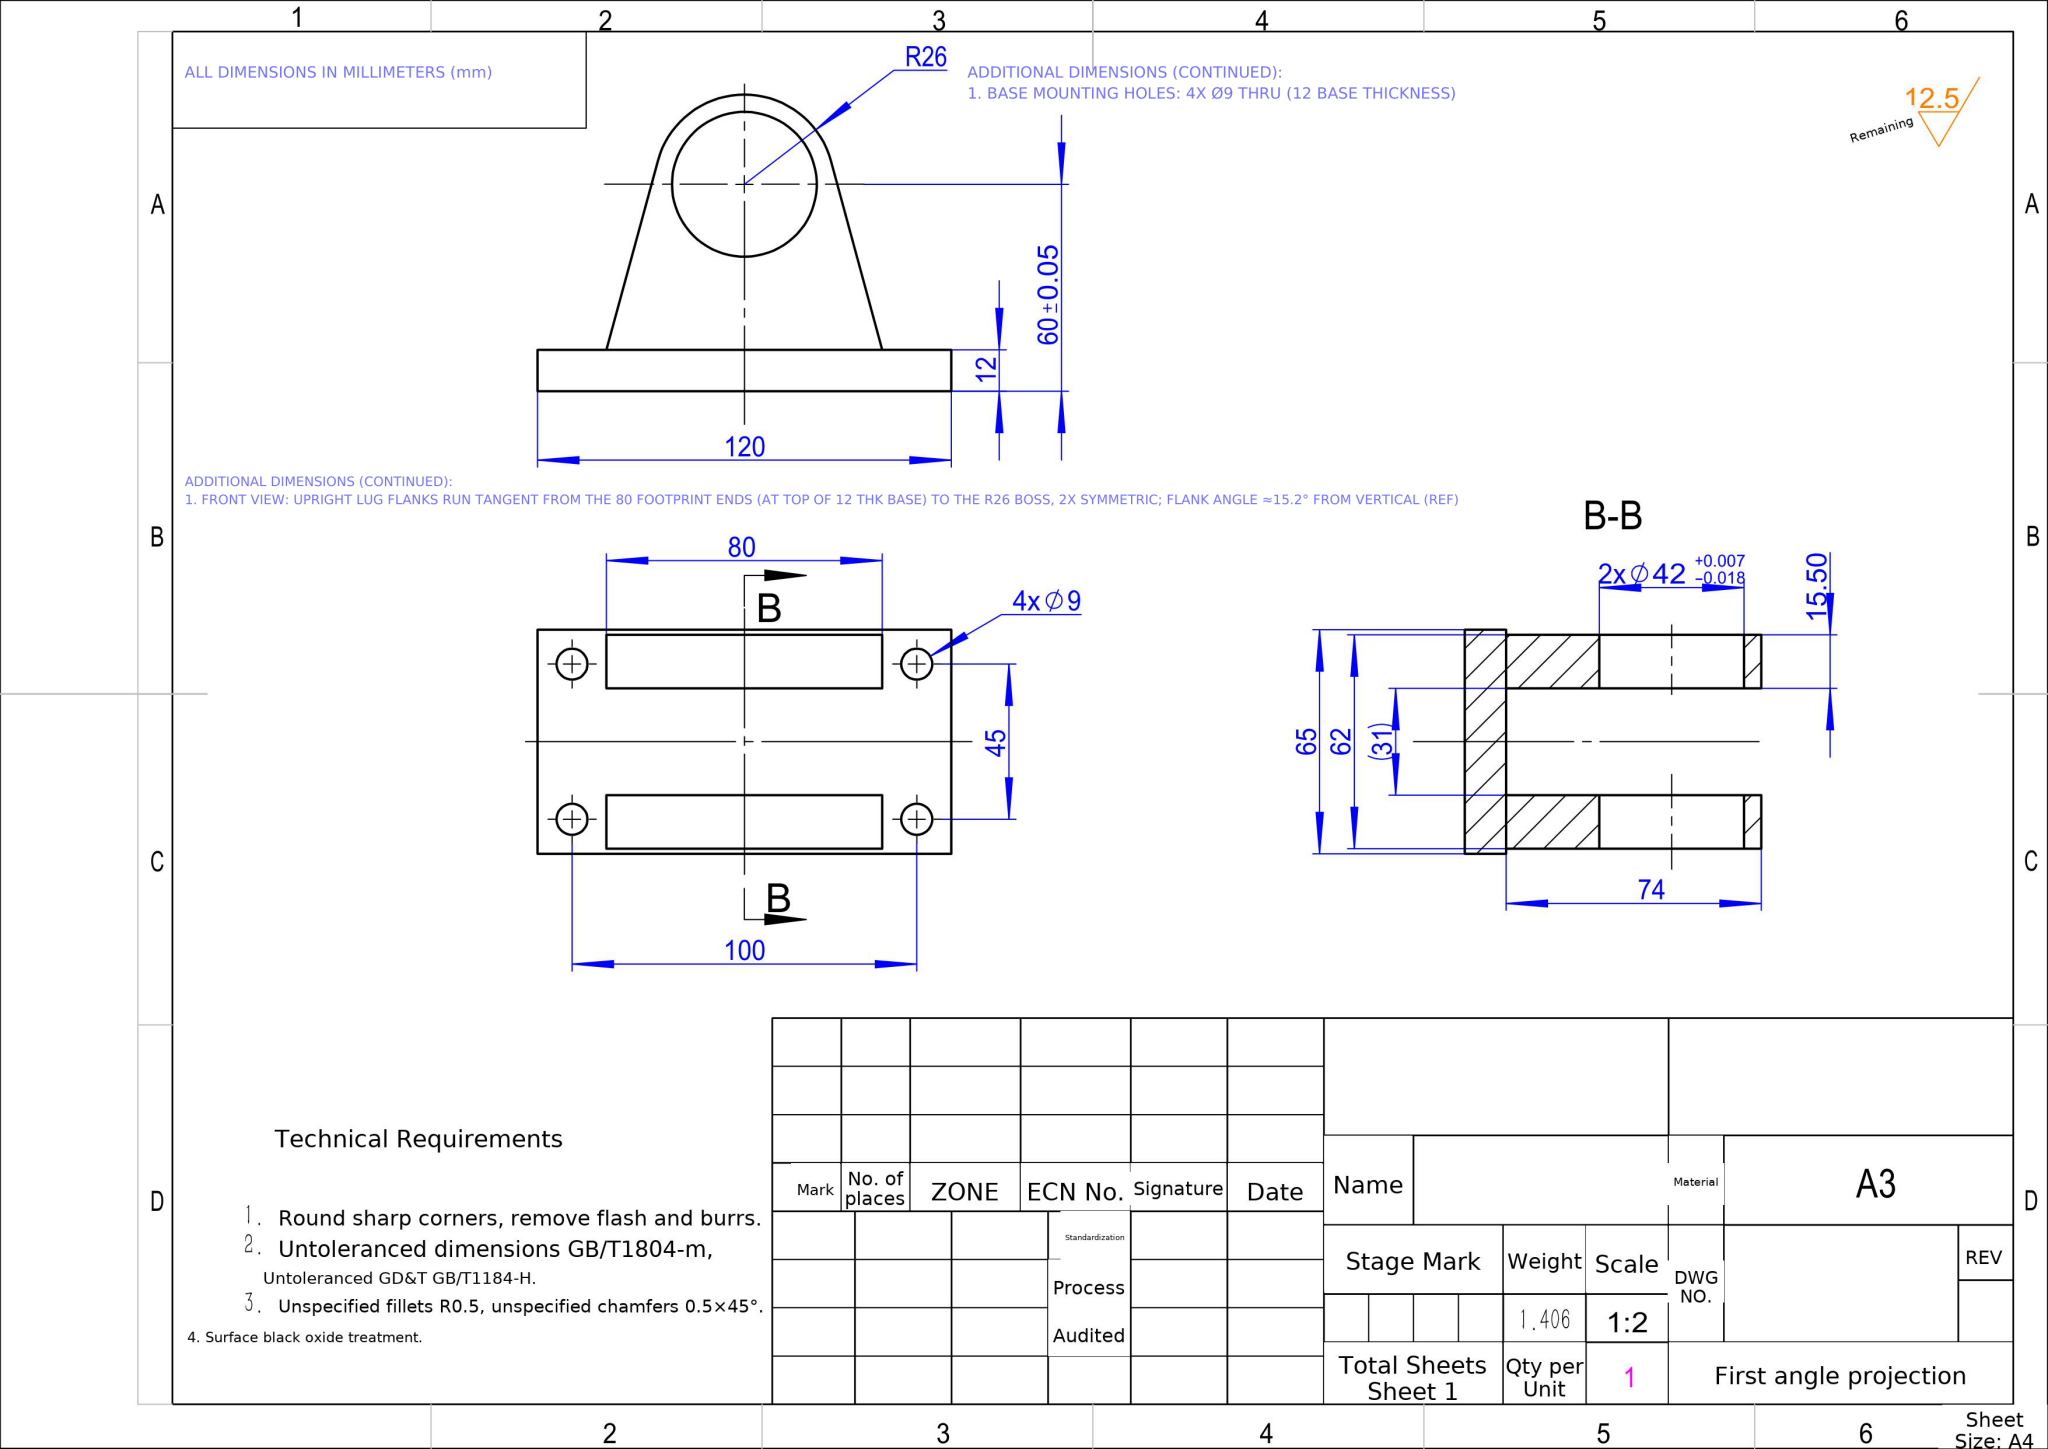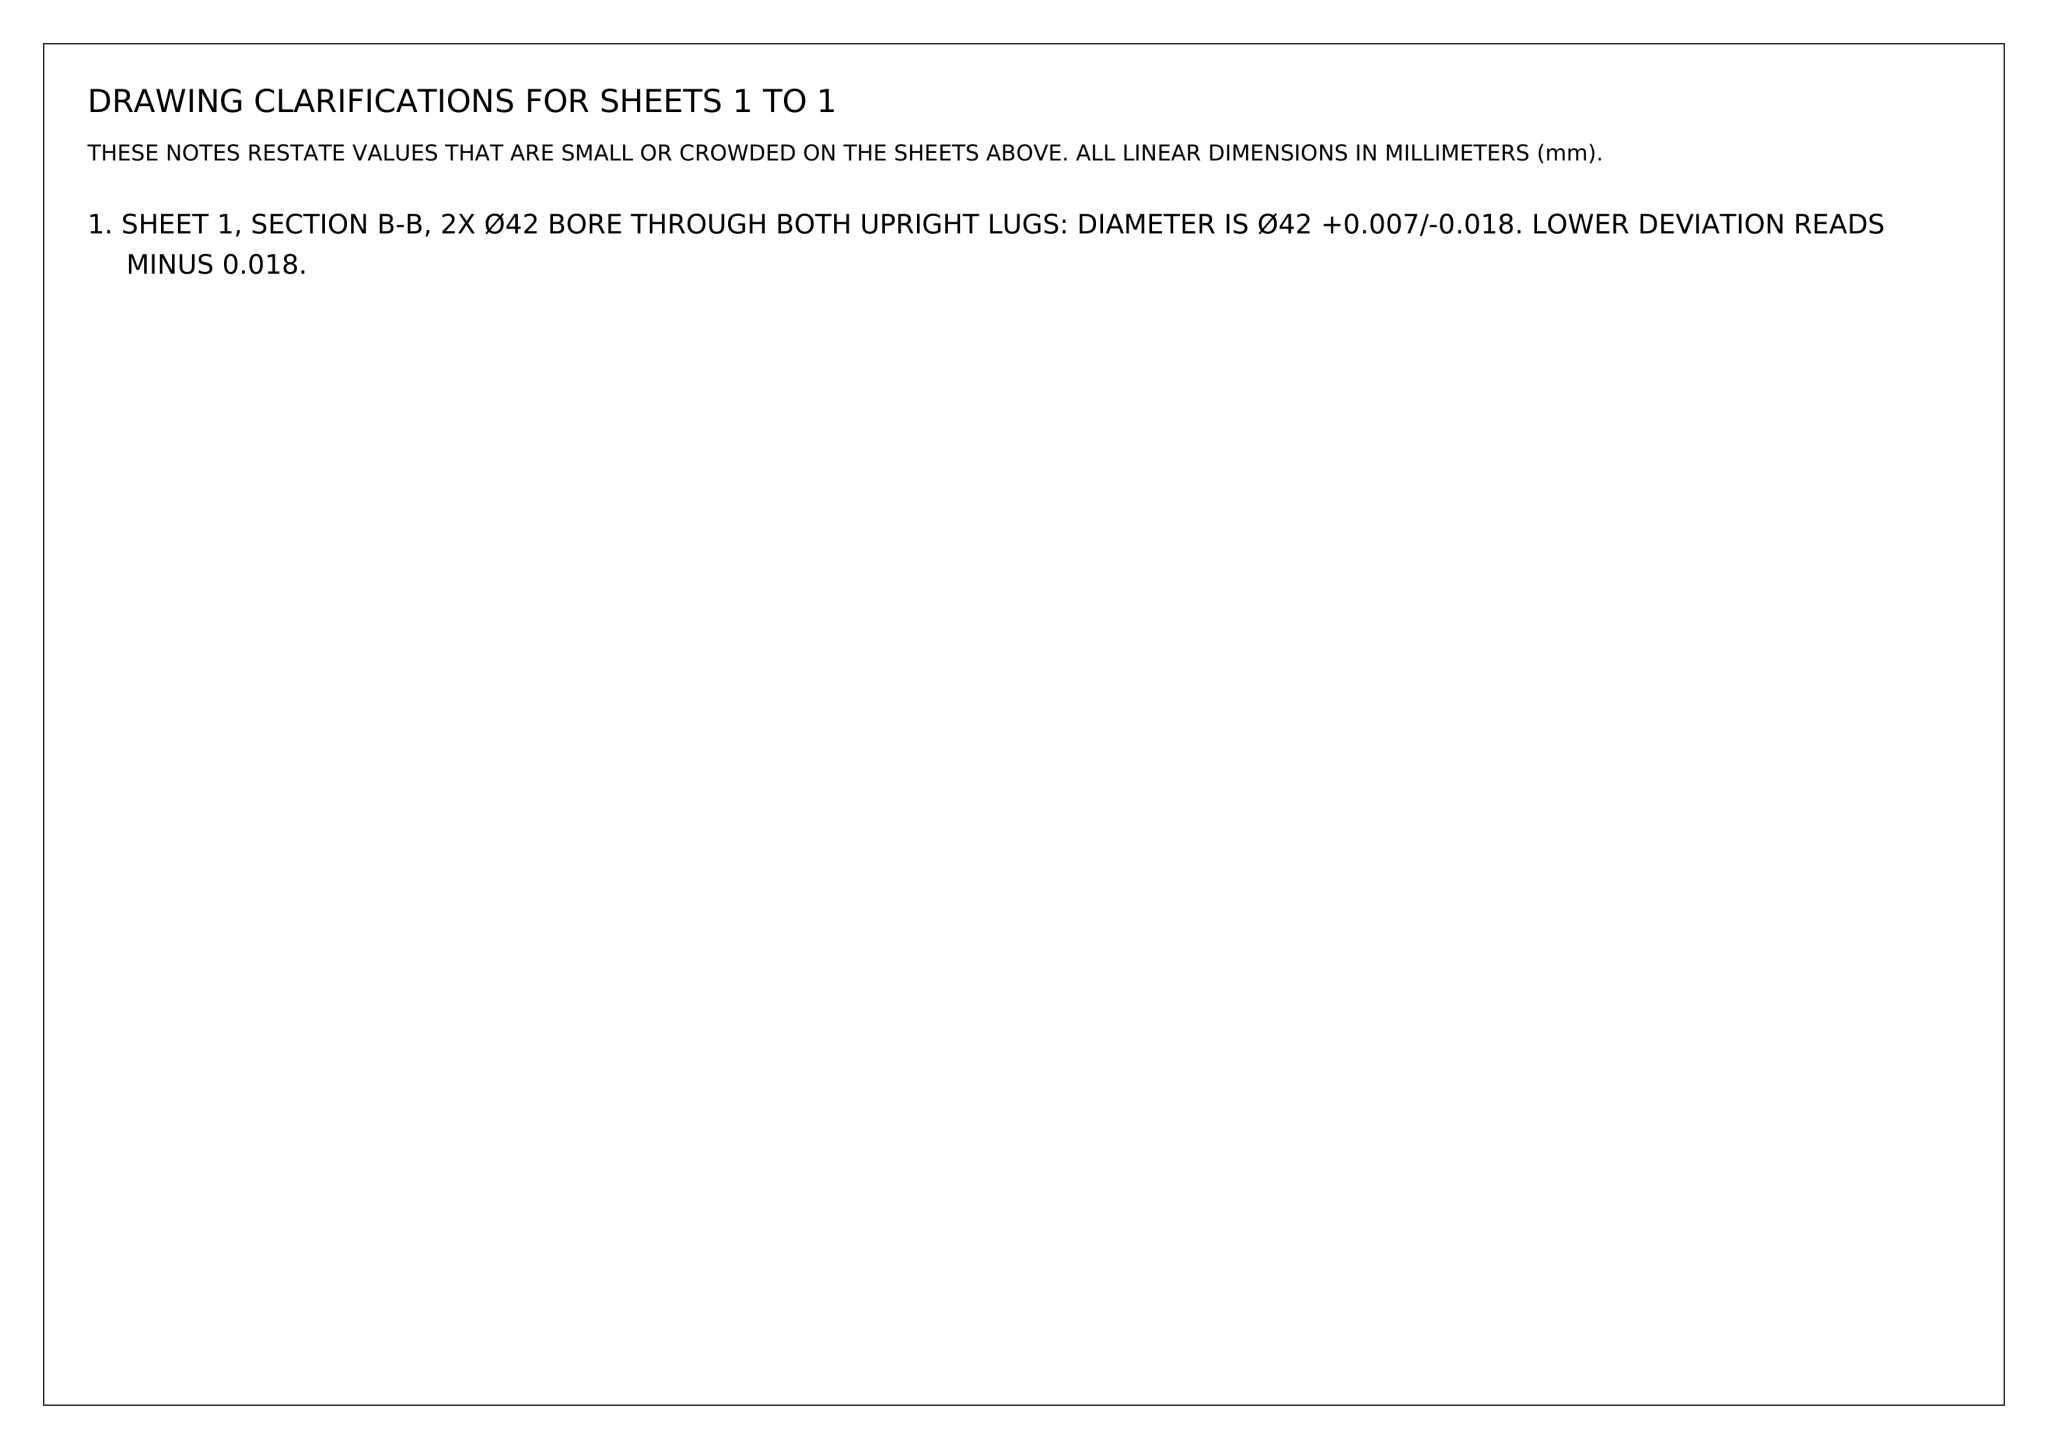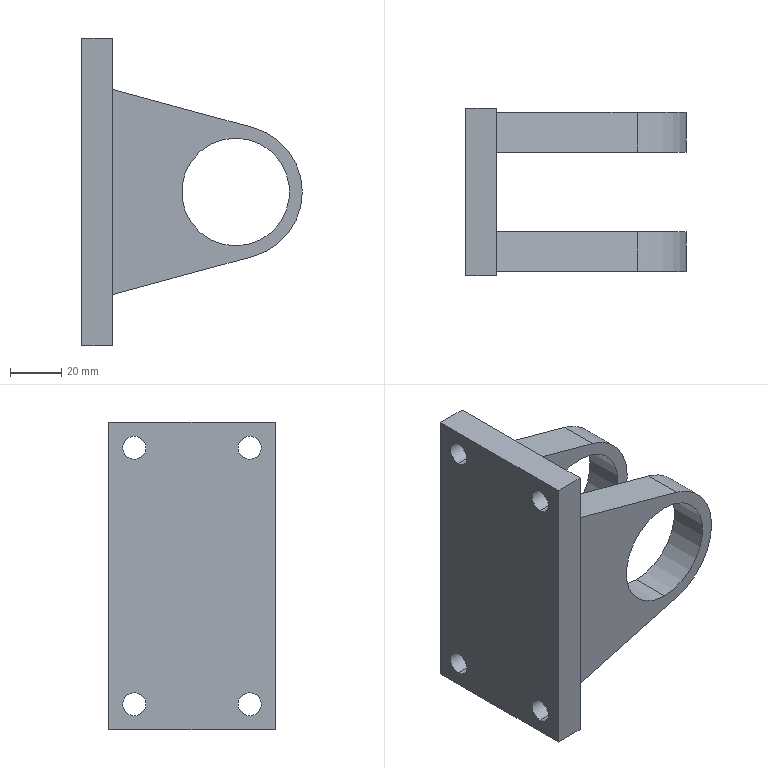Part | NX | mm | 1 solid | 28 faces | box 86 x 65 x 120 mm | volume 180263 mm3 | cylinder 14 | plane 14 | commonest cylinder face diameters 9 x8 42 x4 52 x2
STEP:
#1=COLOUR_RGB('',0.7922,0.8196,0.9333);
#2=FILL_AREA_STYLE_COLOUR('',#1);
#3=FILL_AREA_STYLE('',(#2));
#4=SURFACE_STYLE_FILL_AREA(#3);
#5=SURFACE_SIDE_STYLE('',(#4));
#6=SURFACE_STYLE_USAGE(.BOTH.,#5);
#7=PRESENTATION_STYLE_ASSIGNMENT((#6));
#8=CARTESIAN_POINT('',(60.,-15.5,-21.));
#9=VERTEX_POINT('',#8);
#10=CARTESIAN_POINT('',(60.,-31.,-21.));
#11=VERTEX_POINT('',#10);
#12=CARTESIAN_POINT('',(60.,32.5,-21.));
#13=DIRECTION('',(0.,-1.,0.));
#14=VECTOR('',#13,1000.);
#15=LINE('',#12,#14);
#16=EDGE_CURVE('',#9,#11,#15,.T.);
#17=ORIENTED_EDGE('',*,*,#16,.F.);
#18=CARTESIAN_POINT('',(60.,-15.5,21.));
#19=VERTEX_POINT('',#18);
#20=CARTESIAN_POINT('',(60.,-15.5,0.));
#21=DIRECTION('',(0.,-1.,0.));
#22=DIRECTION('',(0.,0.,-1.));
#23=AXIS2_PLACEMENT_3D('',#20,#21,#22);
#24=CIRCLE('',#23,21.);
#25=EDGE_CURVE('',#19,#9,#24,.T.);
#26=ORIENTED_EDGE('',*,*,#25,.F.);
#27=CARTESIAN_POINT('',(60.,-31.,21.));
#28=VERTEX_POINT('',#27);
#29=CARTESIAN_POINT('',(60.,32.5,21.));
#30=DIRECTION('',(0.,-1.,0.));
#31=VECTOR('',#30,1000.);
#32=LINE('',#29,#31);
#33=EDGE_CURVE('',#19,#28,#32,.T.);
#34=ORIENTED_EDGE('',*,*,#33,.T.);
#35=CARTESIAN_POINT('',(60.,-31.,0.));
#36=DIRECTION('',(0.,1.,0.));
#37=DIRECTION('',(0.,0.,1.));
#38=AXIS2_PLACEMENT_3D('',#35,#36,#37);
#39=CIRCLE('',#38,21.);
#40=EDGE_CURVE('',#11,#28,#39,.T.);
#41=ORIENTED_EDGE('',*,*,#40,.F.);
#42=EDGE_LOOP('',(#17,#26,#34,#41));
#43=FACE_OUTER_BOUND('',#42,.T.);
#44=CARTESIAN_POINT('',(60.,32.5,0.));
#45=DIRECTION('',(0.,-1.,0.));
#46=DIRECTION('',(0.,0.,1.));
#47=AXIS2_PLACEMENT_3D('',#44,#45,#46);
#48=CYLINDRICAL_SURFACE('',#47,21.);
#49=ADVANCED_FACE('',(#43),#48,.F.);
#50=CARTESIAN_POINT('',(66.824,-15.5,-25.089));
#51=VERTEX_POINT('',#50);
#52=CARTESIAN_POINT('',(12.,-15.5,-40.));
#53=VERTEX_POINT('',#52);
#54=CARTESIAN_POINT('',(12.,-15.5,-40.));
#55=DIRECTION('',(-0.9649,0.,-0.2625));
#56=VECTOR('',#55,1000.);
#57=LINE('',#54,#56);
#58=EDGE_CURVE('',#51,#53,#57,.T.);
#59=ORIENTED_EDGE('',*,*,#58,.F.);
#60=CARTESIAN_POINT('',(66.824,-31.,-25.089));
#61=VERTEX_POINT('',#60);
#62=CARTESIAN_POINT('',(66.824,-31.,-25.089));
#63=DIRECTION('',(0.,1.,0.));
#64=VECTOR('',#63,1000.);
#65=LINE('',#62,#64);
#66=EDGE_CURVE('',#61,#51,#65,.T.);
#67=ORIENTED_EDGE('',*,*,#66,.F.);
#68=CARTESIAN_POINT('',(12.,-31.,-40.));
#69=VERTEX_POINT('',#68);
#70=CARTESIAN_POINT('',(12.,-31.,-40.));
#71=DIRECTION('',(-0.9649,0.,-0.2625));
#72=VECTOR('',#71,1000.);
#73=LINE('',#70,#72);
#74=EDGE_CURVE('',#61,#69,#73,.T.);
#75=ORIENTED_EDGE('',*,*,#74,.T.);
#76=CARTESIAN_POINT('',(12.,-31.,-40.));
#77=DIRECTION('',(0.,1.,0.));
#78=VECTOR('',#77,1000.);
#79=LINE('',#76,#78);
#80=EDGE_CURVE('',#69,#53,#79,.T.);
#81=ORIENTED_EDGE('',*,*,#80,.T.);
#82=EDGE_LOOP('',(#59,#67,#75,#81));
#83=FACE_OUTER_BOUND('',#82,.T.);
#84=CARTESIAN_POINT('',(12.,-31.,-40.));
#85=DIRECTION('',(-0.2625,0.,0.9649));
#86=DIRECTION('',(0.,1.,0.));
#87=AXIS2_PLACEMENT_3D('',#84,#85,#86);
#88=PLANE('',#87);
#89=ADVANCED_FACE('',(#83),#88,.F.);
#90=CARTESIAN_POINT('',(66.824,-15.5,25.089));
#91=VERTEX_POINT('',#90);
#92=CARTESIAN_POINT('',(60.,-15.5,0.));
#93=DIRECTION('',(0.,1.,0.));
#94=DIRECTION('',(0.,0.,-1.));
#95=AXIS2_PLACEMENT_3D('',#92,#93,#94);
#96=CIRCLE('',#95,26.);
#97=EDGE_CURVE('',#91,#51,#96,.T.);
#98=ORIENTED_EDGE('',*,*,#97,.F.);
#99=CARTESIAN_POINT('',(66.824,-31.,25.089));
#100=VERTEX_POINT('',#99);
#101=CARTESIAN_POINT('',(66.824,-31.,25.089));
#102=DIRECTION('',(0.,1.,0.));
#103=VECTOR('',#102,1000.);
#104=LINE('',#101,#103);
#105=EDGE_CURVE('',#100,#91,#104,.T.);
#106=ORIENTED_EDGE('',*,*,#105,.F.);
#107=CARTESIAN_POINT('',(60.,-31.,0.));
#108=DIRECTION('',(0.,1.,0.));
#109=DIRECTION('',(0.,0.,-1.));
#110=AXIS2_PLACEMENT_3D('',#107,#108,#109);
#111=CIRCLE('',#110,26.);
#112=EDGE_CURVE('',#100,#61,#111,.T.);
#113=ORIENTED_EDGE('',*,*,#112,.T.);
#114=ORIENTED_EDGE('',*,*,#66,.T.);
#115=EDGE_LOOP('',(#98,#106,#113,#114));
#116=FACE_OUTER_BOUND('',#115,.T.);
#117=CARTESIAN_POINT('',(60.,-31.,0.));
#118=DIRECTION('',(0.,1.,0.));
#119=DIRECTION('',(0.,0.,-1.));
#120=AXIS2_PLACEMENT_3D('',#117,#118,#119);
#121=CYLINDRICAL_SURFACE('',#120,26.);
#122=ADVANCED_FACE('',(#116),#121,.T.);
#123=CARTESIAN_POINT('',(12.,-15.5,40.));
#124=VERTEX_POINT('',#123);
#125=CARTESIAN_POINT('',(66.824,-15.5,25.089));
#126=DIRECTION('',(0.9649,0.,-0.2625));
#127=VECTOR('',#126,1000.);
#128=LINE('',#125,#127);
#129=EDGE_CURVE('',#124,#91,#128,.T.);
#130=ORIENTED_EDGE('',*,*,#129,.F.);
#131=CARTESIAN_POINT('',(12.,-31.,40.));
#132=VERTEX_POINT('',#131);
#133=CARTESIAN_POINT('',(12.,-31.,40.));
#134=DIRECTION('',(0.,1.,0.));
#135=VECTOR('',#134,1000.);
#136=LINE('',#133,#135);
#137=EDGE_CURVE('',#132,#124,#136,.T.);
#138=ORIENTED_EDGE('',*,*,#137,.F.);
#139=CARTESIAN_POINT('',(66.824,-31.,25.089));
#140=DIRECTION('',(0.9649,0.,-0.2625));
#141=VECTOR('',#140,1000.);
#142=LINE('',#139,#141);
#143=EDGE_CURVE('',#132,#100,#142,.T.);
#144=ORIENTED_EDGE('',*,*,#143,.T.);
#145=ORIENTED_EDGE('',*,*,#105,.T.);
#146=EDGE_LOOP('',(#130,#138,#144,#145));
#147=FACE_OUTER_BOUND('',#146,.T.);
#148=CARTESIAN_POINT('',(66.824,-31.,25.089));
#149=DIRECTION('',(-0.2625,0.,-0.9649));
#150=DIRECTION('',(-0.9649,0.,0.2625));
#151=AXIS2_PLACEMENT_3D('',#148,#149,#150);
#152=PLANE('',#151);
#153=ADVANCED_FACE('',(#147),#152,.F.);
#154=ORIENTED_EDGE('',*,*,#25,.T.);
#155=CARTESIAN_POINT('',(60.,-15.5,0.));
#156=DIRECTION('',(0.,-1.,0.));
#157=DIRECTION('',(0.,0.,-1.));
#158=AXIS2_PLACEMENT_3D('',#155,#156,#157);
#159=CIRCLE('',#158,21.);
#160=EDGE_CURVE('',#9,#19,#159,.T.);
#161=ORIENTED_EDGE('',*,*,#160,.T.);
#162=EDGE_LOOP('',(#154,#161));
#163=FACE_BOUND('',#162,.T.);
#164=CARTESIAN_POINT('',(12.,-15.5,40.));
#165=DIRECTION('',(0.,0.,1.));
#166=VECTOR('',#165,1000.);
#167=LINE('',#164,#166);
#168=EDGE_CURVE('',#53,#124,#167,.T.);
#169=ORIENTED_EDGE('',*,*,#168,.T.);
#170=ORIENTED_EDGE('',*,*,#129,.T.);
#171=ORIENTED_EDGE('',*,*,#97,.T.);
#172=ORIENTED_EDGE('',*,*,#58,.T.);
#173=EDGE_LOOP('',(#169,#170,#171,#172));
#174=FACE_OUTER_BOUND('',#173,.T.);
#175=CARTESIAN_POINT('',(60.,-15.5,0.));
#176=DIRECTION('',(0.,1.,0.));
#177=DIRECTION('',(1.,0.,0.));
#178=AXIS2_PLACEMENT_3D('',#175,#176,#177);
#179=PLANE('',#178);
#180=ADVANCED_FACE('',(#163,#174),#179,.T.);
#181=CARTESIAN_POINT('',(60.,-31.,0.));
#182=DIRECTION('',(0.,1.,0.));
#183=DIRECTION('',(0.,0.,1.));
#184=AXIS2_PLACEMENT_3D('',#181,#182,#183);
#185=CIRCLE('',#184,21.);
#186=EDGE_CURVE('',#28,#11,#185,.T.);
#187=ORIENTED_EDGE('',*,*,#186,.T.);
#188=ORIENTED_EDGE('',*,*,#40,.T.);
#189=EDGE_LOOP('',(#187,#188));
#190=FACE_BOUND('',#189,.T.);
#191=CARTESIAN_POINT('',(12.,-31.,40.));
#192=DIRECTION('',(0.,0.,1.));
#193=VECTOR('',#192,1000.);
#194=LINE('',#191,#193);
#195=EDGE_CURVE('',#69,#132,#194,.T.);
#196=ORIENTED_EDGE('',*,*,#195,.F.);
#197=ORIENTED_EDGE('',*,*,#74,.F.);
#198=ORIENTED_EDGE('',*,*,#112,.F.);
#199=ORIENTED_EDGE('',*,*,#143,.F.);
#200=EDGE_LOOP('',(#196,#197,#198,#199));
#201=FACE_OUTER_BOUND('',#200,.T.);
#202=CARTESIAN_POINT('',(60.,-31.,0.));
#203=DIRECTION('',(0.,1.,0.));
#204=DIRECTION('',(1.,0.,0.));
#205=AXIS2_PLACEMENT_3D('',#202,#203,#204);
#206=PLANE('',#205);
#207=ADVANCED_FACE('',(#190,#201),#206,.F.);
#208=ORIENTED_EDGE('',*,*,#160,.F.);
#209=ORIENTED_EDGE('',*,*,#16,.T.);
#210=ORIENTED_EDGE('',*,*,#186,.F.);
#211=ORIENTED_EDGE('',*,*,#33,.F.);
#212=EDGE_LOOP('',(#208,#209,#210,#211));
#213=FACE_OUTER_BOUND('',#212,.T.);
#214=CARTESIAN_POINT('',(60.,32.5,0.));
#215=DIRECTION('',(0.,-1.,0.));
#216=DIRECTION('',(0.,0.,1.));
#217=AXIS2_PLACEMENT_3D('',#214,#215,#216);
#218=CYLINDRICAL_SURFACE('',#217,21.);
#219=ADVANCED_FACE('',(#213),#218,.F.);
#220=CARTESIAN_POINT('',(12.,31.,-40.));
#221=VERTEX_POINT('',#220);
#222=CARTESIAN_POINT('',(12.,15.5,-40.));
#223=VERTEX_POINT('',#222);
#224=CARTESIAN_POINT('',(12.,31.,-40.));
#225=DIRECTION('',(0.,-1.,0.));
#226=VECTOR('',#225,1000.);
#227=LINE('',#224,#226);
#228=EDGE_CURVE('',#221,#223,#227,.T.);
#229=ORIENTED_EDGE('',*,*,#228,.T.);
#230=CARTESIAN_POINT('',(12.,15.5,40.));
#231=VERTEX_POINT('',#230);
#232=CARTESIAN_POINT('',(12.,15.5,40.));
#233=DIRECTION('',(0.,0.,1.));
#234=VECTOR('',#233,1000.);
#235=LINE('',#232,#234);
#236=EDGE_CURVE('',#223,#231,#235,.T.);
#237=ORIENTED_EDGE('',*,*,#236,.T.);
#238=CARTESIAN_POINT('',(12.,31.,40.));
#239=VERTEX_POINT('',#238);
#240=CARTESIAN_POINT('',(12.,31.,40.));
#241=DIRECTION('',(0.,-1.,0.));
#242=VECTOR('',#241,1000.);
#243=LINE('',#240,#242);
#244=EDGE_CURVE('',#239,#231,#243,.T.);
#245=ORIENTED_EDGE('',*,*,#244,.F.);
#246=CARTESIAN_POINT('',(12.,31.,40.));
#247=DIRECTION('',(0.,0.,1.));
#248=VECTOR('',#247,1000.);
#249=LINE('',#246,#248);
#250=EDGE_CURVE('',#221,#239,#249,.T.);
#251=ORIENTED_EDGE('',*,*,#250,.F.);
#252=EDGE_LOOP('',(#229,#237,#245,#251));
#253=FACE_BOUND('',#252,.T.);
#254=CARTESIAN_POINT('',(12.,-32.5,-60.));
#255=VERTEX_POINT('',#254);
#256=CARTESIAN_POINT('',(12.,32.5,-60.));
#257=VERTEX_POINT('',#256);
#258=CARTESIAN_POINT('',(12.,32.5,-60.));
#259=DIRECTION('',(0.,1.,0.));
#260=VECTOR('',#259,1000.);
#261=LINE('',#258,#260);
#262=EDGE_CURVE('',#255,#257,#261,.T.);
#263=ORIENTED_EDGE('',*,*,#262,.T.);
#264=CARTESIAN_POINT('',(12.,32.5,60.));
#265=VERTEX_POINT('',#264);
#266=CARTESIAN_POINT('',(12.,32.5,60.));
#267=DIRECTION('',(0.,0.,1.));
#268=VECTOR('',#267,1000.);
#269=LINE('',#266,#268);
#270=EDGE_CURVE('',#257,#265,#269,.T.);
#271=ORIENTED_EDGE('',*,*,#270,.T.);
#272=CARTESIAN_POINT('',(12.,-32.5,60.));
#273=VERTEX_POINT('',#272);
#274=CARTESIAN_POINT('',(12.,32.5,60.));
#275=DIRECTION('',(0.,-1.,0.));
#276=VECTOR('',#275,1000.);
#277=LINE('',#274,#276);
#278=EDGE_CURVE('',#265,#273,#277,.T.);
#279=ORIENTED_EDGE('',*,*,#278,.T.);
#280=CARTESIAN_POINT('',(12.,-32.5,60.));
#281=DIRECTION('',(0.,0.,-1.));
#282=VECTOR('',#281,1000.);
#283=LINE('',#280,#282);
#284=EDGE_CURVE('',#273,#255,#283,.T.);
#285=ORIENTED_EDGE('',*,*,#284,.T.);
#286=EDGE_LOOP('',(#263,#271,#279,#285));
#287=FACE_OUTER_BOUND('',#286,.T.);
#288=CARTESIAN_POINT('',(12.,22.5,45.5));
#289=VERTEX_POINT('',#288);
#290=CARTESIAN_POINT('',(12.,22.5,54.5));
#291=VERTEX_POINT('',#290);
#292=CARTESIAN_POINT('',(12.,22.5,50.));
#293=DIRECTION('',(1.,0.,0.));
#294=DIRECTION('',(0.,0.,-1.));
#295=AXIS2_PLACEMENT_3D('',#292,#293,#294);
#296=CIRCLE('',#295,4.5);
#297=EDGE_CURVE('',#289,#291,#296,.T.);
#298=ORIENTED_EDGE('',*,*,#297,.F.);
#299=CARTESIAN_POINT('',(12.,22.5,50.));
#300=DIRECTION('',(1.,0.,0.));
#301=DIRECTION('',(0.,0.,-1.));
#302=AXIS2_PLACEMENT_3D('',#299,#300,#301);
#303=CIRCLE('',#302,4.5);
#304=EDGE_CURVE('',#291,#289,#303,.T.);
#305=ORIENTED_EDGE('',*,*,#304,.F.);
#306=EDGE_LOOP('',(#298,#305));
#307=FACE_BOUND('',#306,.T.);
#308=CARTESIAN_POINT('',(12.,-22.5,45.5));
#309=VERTEX_POINT('',#308);
#310=CARTESIAN_POINT('',(12.,-22.5,54.5));
#311=VERTEX_POINT('',#310);
#312=CARTESIAN_POINT('',(12.,-22.5,50.));
#313=DIRECTION('',(1.,0.,0.));
#314=DIRECTION('',(0.,0.,-1.));
#315=AXIS2_PLACEMENT_3D('',#312,#313,#314);
#316=CIRCLE('',#315,4.5);
#317=EDGE_CURVE('',#309,#311,#316,.T.);
#318=ORIENTED_EDGE('',*,*,#317,.F.);
#319=CARTESIAN_POINT('',(12.,-22.5,50.));
#320=DIRECTION('',(1.,0.,0.));
#321=DIRECTION('',(0.,0.,-1.));
#322=AXIS2_PLACEMENT_3D('',#319,#320,#321);
#323=CIRCLE('',#322,4.5);
#324=EDGE_CURVE('',#311,#309,#323,.T.);
#325=ORIENTED_EDGE('',*,*,#324,.F.);
#326=EDGE_LOOP('',(#318,#325));
#327=FACE_BOUND('',#326,.T.);
#328=CARTESIAN_POINT('',(12.,-22.5,-54.5));
#329=VERTEX_POINT('',#328);
#330=CARTESIAN_POINT('',(12.,-22.5,-45.5));
#331=VERTEX_POINT('',#330);
#332=CARTESIAN_POINT('',(12.,-22.5,-50.));
#333=DIRECTION('',(1.,0.,0.));
#334=DIRECTION('',(0.,0.,-1.));
#335=AXIS2_PLACEMENT_3D('',#332,#333,#334);
#336=CIRCLE('',#335,4.5);
#337=EDGE_CURVE('',#329,#331,#336,.T.);
#338=ORIENTED_EDGE('',*,*,#337,.F.);
#339=CARTESIAN_POINT('',(12.,-22.5,-50.));
#340=DIRECTION('',(1.,0.,0.));
#341=DIRECTION('',(0.,0.,-1.));
#342=AXIS2_PLACEMENT_3D('',#339,#340,#341);
#343=CIRCLE('',#342,4.5);
#344=EDGE_CURVE('',#331,#329,#343,.T.);
#345=ORIENTED_EDGE('',*,*,#344,.F.);
#346=EDGE_LOOP('',(#338,#345));
#347=FACE_BOUND('',#346,.T.);
#348=CARTESIAN_POINT('',(12.,22.5,-54.5));
#349=VERTEX_POINT('',#348);
#350=CARTESIAN_POINT('',(12.,22.5,-45.5));
#351=VERTEX_POINT('',#350);
#352=CARTESIAN_POINT('',(12.,22.5,-50.));
#353=DIRECTION('',(1.,0.,0.));
#354=DIRECTION('',(0.,0.,-1.));
#355=AXIS2_PLACEMENT_3D('',#352,#353,#354);
#356=CIRCLE('',#355,4.5);
#357=EDGE_CURVE('',#349,#351,#356,.T.);
#358=ORIENTED_EDGE('',*,*,#357,.F.);
#359=CARTESIAN_POINT('',(12.,22.5,-50.));
#360=DIRECTION('',(1.,0.,0.));
#361=DIRECTION('',(0.,0.,-1.));
#362=AXIS2_PLACEMENT_3D('',#359,#360,#361);
#363=CIRCLE('',#362,4.5);
#364=EDGE_CURVE('',#351,#349,#363,.T.);
#365=ORIENTED_EDGE('',*,*,#364,.F.);
#366=EDGE_LOOP('',(#358,#365));
#367=FACE_BOUND('',#366,.T.);
#368=ORIENTED_EDGE('',*,*,#168,.F.);
#369=ORIENTED_EDGE('',*,*,#80,.F.);
#370=ORIENTED_EDGE('',*,*,#195,.T.);
#371=ORIENTED_EDGE('',*,*,#137,.T.);
#372=EDGE_LOOP('',(#368,#369,#370,#371));
#373=FACE_BOUND('',#372,.T.);
#374=CARTESIAN_POINT('',(12.,0.,0.));
#375=DIRECTION('',(1.,0.,0.));
#376=DIRECTION('',(0.,1.,0.));
#377=AXIS2_PLACEMENT_3D('',#374,#375,#376);
#378=PLANE('',#377);
#379=ADVANCED_FACE('',(#253,#287,#307,#327,#347,#367,#373),#378,.T.);
#380=CARTESIAN_POINT('',(0.,22.5,54.5));
#381=VERTEX_POINT('',#380);
#382=CARTESIAN_POINT('',(12.,22.5,54.5));
#383=DIRECTION('',(1.,0.,0.));
#384=VECTOR('',#383,1000.);
#385=LINE('',#382,#384);
#386=EDGE_CURVE('',#381,#291,#385,.T.);
#387=ORIENTED_EDGE('',*,*,#386,.F.);
#388=CARTESIAN_POINT('',(0.,22.5,45.5));
#389=VERTEX_POINT('',#388);
#390=CARTESIAN_POINT('',(0.,22.5,50.));
#391=DIRECTION('',(1.,0.,0.));
#392=DIRECTION('',(0.,0.,-1.));
#393=AXIS2_PLACEMENT_3D('',#390,#391,#392);
#394=CIRCLE('',#393,4.5);
#395=EDGE_CURVE('',#389,#381,#394,.T.);
#396=ORIENTED_EDGE('',*,*,#395,.F.);
#397=CARTESIAN_POINT('',(12.,22.5,45.5));
#398=DIRECTION('',(1.,0.,0.));
#399=VECTOR('',#398,1000.);
#400=LINE('',#397,#399);
#401=EDGE_CURVE('',#389,#289,#400,.T.);
#402=ORIENTED_EDGE('',*,*,#401,.T.);
#403=ORIENTED_EDGE('',*,*,#297,.T.);
#404=EDGE_LOOP('',(#387,#396,#402,#403));
#405=FACE_OUTER_BOUND('',#404,.T.);
#406=CARTESIAN_POINT('',(12.,22.5,50.));
#407=DIRECTION('',(1.,0.,0.));
#408=DIRECTION('',(0.,0.,-1.));
#409=AXIS2_PLACEMENT_3D('',#406,#407,#408);
#410=CYLINDRICAL_SURFACE('',#409,4.5);
#411=ADVANCED_FACE('',(#405),#410,.F.);
#412=CARTESIAN_POINT('',(0.,-22.5,54.5));
#413=VERTEX_POINT('',#412);
#414=CARTESIAN_POINT('',(12.,-22.5,54.5));
#415=DIRECTION('',(1.,0.,0.));
#416=VECTOR('',#415,1000.);
#417=LINE('',#414,#416);
#418=EDGE_CURVE('',#413,#311,#417,.T.);
#419=ORIENTED_EDGE('',*,*,#418,.F.);
#420=CARTESIAN_POINT('',(0.,-22.5,45.5));
#421=VERTEX_POINT('',#420);
#422=CARTESIAN_POINT('',(0.,-22.5,50.));
#423=DIRECTION('',(1.,0.,0.));
#424=DIRECTION('',(0.,0.,-1.));
#425=AXIS2_PLACEMENT_3D('',#422,#423,#424);
#426=CIRCLE('',#425,4.5);
#427=EDGE_CURVE('',#421,#413,#426,.T.);
#428=ORIENTED_EDGE('',*,*,#427,.F.);
#429=CARTESIAN_POINT('',(12.,-22.5,45.5));
#430=DIRECTION('',(1.,0.,0.));
#431=VECTOR('',#430,1000.);
#432=LINE('',#429,#431);
#433=EDGE_CURVE('',#421,#309,#432,.T.);
#434=ORIENTED_EDGE('',*,*,#433,.T.);
#435=ORIENTED_EDGE('',*,*,#317,.T.);
#436=EDGE_LOOP('',(#419,#428,#434,#435));
#437=FACE_OUTER_BOUND('',#436,.T.);
#438=CARTESIAN_POINT('',(12.,-22.5,50.));
#439=DIRECTION('',(1.,0.,0.));
#440=DIRECTION('',(0.,0.,-1.));
#441=AXIS2_PLACEMENT_3D('',#438,#439,#440);
#442=CYLINDRICAL_SURFACE('',#441,4.5);
#443=ADVANCED_FACE('',(#437),#442,.F.);
#444=CARTESIAN_POINT('',(0.,-22.5,-45.5));
#445=VERTEX_POINT('',#444);
#446=CARTESIAN_POINT('',(12.,-22.5,-45.5));
#447=DIRECTION('',(1.,0.,0.));
#448=VECTOR('',#447,1000.);
#449=LINE('',#446,#448);
#450=EDGE_CURVE('',#445,#331,#449,.T.);
#451=ORIENTED_EDGE('',*,*,#450,.F.);
#452=CARTESIAN_POINT('',(0.,-22.5,-54.5));
#453=VERTEX_POINT('',#452);
#454=CARTESIAN_POINT('',(0.,-22.5,-50.));
#455=DIRECTION('',(1.,0.,0.));
#456=DIRECTION('',(0.,0.,-1.));
#457=AXIS2_PLACEMENT_3D('',#454,#455,#456);
#458=CIRCLE('',#457,4.5);
#459=EDGE_CURVE('',#453,#445,#458,.T.);
#460=ORIENTED_EDGE('',*,*,#459,.F.);
#461=CARTESIAN_POINT('',(12.,-22.5,-54.5));
#462=DIRECTION('',(1.,0.,0.));
#463=VECTOR('',#462,1000.);
#464=LINE('',#461,#463);
#465=EDGE_CURVE('',#453,#329,#464,.T.);
#466=ORIENTED_EDGE('',*,*,#465,.T.);
#467=ORIENTED_EDGE('',*,*,#337,.T.);
#468=EDGE_LOOP('',(#451,#460,#466,#467));
#469=FACE_OUTER_BOUND('',#468,.T.);
#470=CARTESIAN_POINT('',(12.,-22.5,-50.));
#471=DIRECTION('',(1.,0.,0.));
#472=DIRECTION('',(0.,0.,-1.));
#473=AXIS2_PLACEMENT_3D('',#470,#471,#472);
#474=CYLINDRICAL_SURFACE('',#473,4.5);
#475=ADVANCED_FACE('',(#469),#474,.F.);
#476=CARTESIAN_POINT('',(0.,22.5,-45.5));
#477=VERTEX_POINT('',#476);
#478=CARTESIAN_POINT('',(12.,22.5,-45.5));
#479=DIRECTION('',(1.,0.,0.));
#480=VECTOR('',#479,1000.);
#481=LINE('',#478,#480);
#482=EDGE_CURVE('',#477,#351,#481,.T.);
#483=ORIENTED_EDGE('',*,*,#482,.F.);
#484=CARTESIAN_POINT('',(0.,22.5,-54.5));
#485=VERTEX_POINT('',#484);
#486=CARTESIAN_POINT('',(0.,22.5,-50.));
#487=DIRECTION('',(1.,0.,0.));
#488=DIRECTION('',(0.,0.,-1.));
#489=AXIS2_PLACEMENT_3D('',#486,#487,#488);
#490=CIRCLE('',#489,4.5);
#491=EDGE_CURVE('',#485,#477,#490,.T.);
#492=ORIENTED_EDGE('',*,*,#491,.F.);
#493=CARTESIAN_POINT('',(12.,22.5,-54.5));
#494=DIRECTION('',(1.,0.,0.));
#495=VECTOR('',#494,1000.);
#496=LINE('',#493,#495);
#497=EDGE_CURVE('',#485,#349,#496,.T.);
#498=ORIENTED_EDGE('',*,*,#497,.T.);
#499=ORIENTED_EDGE('',*,*,#357,.T.);
#500=EDGE_LOOP('',(#483,#492,#498,#499));
#501=FACE_OUTER_BOUND('',#500,.T.);
#502=CARTESIAN_POINT('',(12.,22.5,-50.));
#503=DIRECTION('',(1.,0.,0.));
#504=DIRECTION('',(0.,0.,-1.));
#505=AXIS2_PLACEMENT_3D('',#502,#503,#504);
#506=CYLINDRICAL_SURFACE('',#505,4.5);
#507=ADVANCED_FACE('',(#501),#506,.F.);
#508=ORIENTED_EDGE('',*,*,#491,.T.);
#509=CARTESIAN_POINT('',(0.,22.5,-50.));
#510=DIRECTION('',(1.,0.,0.));
#511=DIRECTION('',(0.,0.,-1.));
#512=AXIS2_PLACEMENT_3D('',#509,#510,#511);
#513=CIRCLE('',#512,4.5);
#514=EDGE_CURVE('',#477,#485,#513,.T.);
#515=ORIENTED_EDGE('',*,*,#514,.T.);
#516=EDGE_LOOP('',(#508,#515));
#517=FACE_BOUND('',#516,.T.);
#518=ORIENTED_EDGE('',*,*,#459,.T.);
#519=CARTESIAN_POINT('',(0.,-22.5,-50.));
#520=DIRECTION('',(1.,0.,0.));
#521=DIRECTION('',(0.,0.,-1.));
#522=AXIS2_PLACEMENT_3D('',#519,#520,#521);
#523=CIRCLE('',#522,4.5);
#524=EDGE_CURVE('',#445,#453,#523,.T.);
#525=ORIENTED_EDGE('',*,*,#524,.T.);
#526=EDGE_LOOP('',(#518,#525));
#527=FACE_BOUND('',#526,.T.);
#528=ORIENTED_EDGE('',*,*,#427,.T.);
#529=CARTESIAN_POINT('',(0.,-22.5,50.));
#530=DIRECTION('',(1.,0.,0.));
#531=DIRECTION('',(0.,0.,-1.));
#532=AXIS2_PLACEMENT_3D('',#529,#530,#531);
#533=CIRCLE('',#532,4.5);
#534=EDGE_CURVE('',#413,#421,#533,.T.);
#535=ORIENTED_EDGE('',*,*,#534,.T.);
#536=EDGE_LOOP('',(#528,#535));
#537=FACE_BOUND('',#536,.T.);
#538=ORIENTED_EDGE('',*,*,#395,.T.);
#539=CARTESIAN_POINT('',(0.,22.5,50.));
#540=DIRECTION('',(1.,0.,0.));
#541=DIRECTION('',(0.,0.,-1.));
#542=AXIS2_PLACEMENT_3D('',#539,#540,#541);
#543=CIRCLE('',#542,4.5);
#544=EDGE_CURVE('',#381,#389,#543,.T.);
#545=ORIENTED_EDGE('',*,*,#544,.T.);
#546=EDGE_LOOP('',(#538,#545));
#547=FACE_BOUND('',#546,.T.);
#548=CARTESIAN_POINT('',(0.,-32.5,-60.));
#549=VERTEX_POINT('',#548);
#550=CARTESIAN_POINT('',(0.,32.5,-60.));
#551=VERTEX_POINT('',#550);
#552=CARTESIAN_POINT('',(0.,32.5,-60.));
#553=DIRECTION('',(0.,1.,0.));
#554=VECTOR('',#553,1000.);
#555=LINE('',#552,#554);
#556=EDGE_CURVE('',#549,#551,#555,.T.);
#557=ORIENTED_EDGE('',*,*,#556,.F.);
#558=CARTESIAN_POINT('',(0.,-32.5,60.));
#559=VERTEX_POINT('',#558);
#560=CARTESIAN_POINT('',(0.,-32.5,60.));
#561=DIRECTION('',(0.,0.,-1.));
#562=VECTOR('',#561,1000.);
#563=LINE('',#560,#562);
#564=EDGE_CURVE('',#559,#549,#563,.T.);
#565=ORIENTED_EDGE('',*,*,#564,.F.);
#566=CARTESIAN_POINT('',(0.,32.5,60.));
#567=VERTEX_POINT('',#566);
#568=CARTESIAN_POINT('',(0.,32.5,60.));
#569=DIRECTION('',(0.,-1.,0.));
#570=VECTOR('',#569,1000.);
#571=LINE('',#568,#570);
#572=EDGE_CURVE('',#567,#559,#571,.T.);
#573=ORIENTED_EDGE('',*,*,#572,.F.);
#574=CARTESIAN_POINT('',(0.,32.5,60.));
#575=DIRECTION('',(0.,0.,1.));
#576=VECTOR('',#575,1000.);
#577=LINE('',#574,#576);
#578=EDGE_CURVE('',#551,#567,#577,.T.);
#579=ORIENTED_EDGE('',*,*,#578,.F.);
#580=EDGE_LOOP('',(#557,#565,#573,#579));
#581=FACE_OUTER_BOUND('',#580,.T.);
#582=CARTESIAN_POINT('',(0.,0.,0.));
#583=DIRECTION('',(1.,0.,0.));
#584=DIRECTION('',(0.,1.,0.));
#585=AXIS2_PLACEMENT_3D('',#582,#583,#584);
#586=PLANE('',#585);
#587=ADVANCED_FACE('',(#517,#527,#537,#547,#581),#586,.F.);
#588=ORIENTED_EDGE('',*,*,#564,.T.);
#589=CARTESIAN_POINT('',(12.,-32.5,-60.));
#590=DIRECTION('',(-1.,0.,0.));
#591=VECTOR('',#590,1000.);
#592=LINE('',#589,#591);
#593=EDGE_CURVE('',#255,#549,#592,.T.);
#594=ORIENTED_EDGE('',*,*,#593,.F.);
#595=ORIENTED_EDGE('',*,*,#284,.F.);
#596=CARTESIAN_POINT('',(12.,-32.5,60.));
#597=DIRECTION('',(-1.,0.,0.));
#598=VECTOR('',#597,1000.);
#599=LINE('',#596,#598);
#600=EDGE_CURVE('',#273,#559,#599,.T.);
#601=ORIENTED_EDGE('',*,*,#600,.T.);
#602=EDGE_LOOP('',(#588,#594,#595,#601));
#603=FACE_OUTER_BOUND('',#602,.T.);
#604=CARTESIAN_POINT('',(12.,-32.5,60.));
#605=DIRECTION('',(0.,1.,0.));
#606=DIRECTION('',(1.,0.,0.));
#607=AXIS2_PLACEMENT_3D('',#604,#605,#606);
#608=PLANE('',#607);
#609=ADVANCED_FACE('',(#603),#608,.F.);
#610=ORIENTED_EDGE('',*,*,#572,.T.);
#611=ORIENTED_EDGE('',*,*,#600,.F.);
#612=ORIENTED_EDGE('',*,*,#278,.F.);
#613=CARTESIAN_POINT('',(12.,32.5,60.));
#614=DIRECTION('',(-1.,0.,0.));
#615=VECTOR('',#614,1000.);
#616=LINE('',#613,#615);
#617=EDGE_CURVE('',#265,#567,#616,.T.);
#618=ORIENTED_EDGE('',*,*,#617,.T.);
#619=EDGE_LOOP('',(#610,#611,#612,#618));
#620=FACE_OUTER_BOUND('',#619,.T.);
#621=CARTESIAN_POINT('',(12.,32.5,60.));
#622=DIRECTION('',(0.,0.,-1.));
#623=DIRECTION('',(0.,-1.,0.));
#624=AXIS2_PLACEMENT_3D('',#621,#622,#623);
#625=PLANE('',#624);
#626=ADVANCED_FACE('',(#620),#625,.F.);
#627=ORIENTED_EDGE('',*,*,#578,.T.);
#628=ORIENTED_EDGE('',*,*,#617,.F.);
#629=ORIENTED_EDGE('',*,*,#270,.F.);
#630=CARTESIAN_POINT('',(12.,32.5,-60.));
#631=DIRECTION('',(-1.,0.,0.));
#632=VECTOR('',#631,1000.);
#633=LINE('',#630,#632);
#634=EDGE_CURVE('',#257,#551,#633,.T.);
#635=ORIENTED_EDGE('',*,*,#634,.T.);
#636=EDGE_LOOP('',(#627,#628,#629,#635));
#637=FACE_OUTER_BOUND('',#636,.T.);
#638=CARTESIAN_POINT('',(12.,32.5,60.));
#639=DIRECTION('',(0.,-1.,0.));
#640=DIRECTION('',(0.,0.,-1.));
#641=AXIS2_PLACEMENT_3D('',#638,#639,#640);
#642=PLANE('',#641);
#643=ADVANCED_FACE('',(#637),#642,.F.);
#644=ORIENTED_EDGE('',*,*,#556,.T.);
#645=ORIENTED_EDGE('',*,*,#634,.F.);
#646=ORIENTED_EDGE('',*,*,#262,.F.);
#647=ORIENTED_EDGE('',*,*,#593,.T.);
#648=EDGE_LOOP('',(#644,#645,#646,#647));
#649=FACE_OUTER_BOUND('',#648,.T.);
#650=CARTESIAN_POINT('',(12.,32.5,-60.));
#651=DIRECTION('',(0.,0.,1.));
#652=DIRECTION('',(1.,0.,0.));
#653=AXIS2_PLACEMENT_3D('',#650,#651,#652);
#654=PLANE('',#653);
#655=ADVANCED_FACE('',(#649),#654,.F.);
#656=ORIENTED_EDGE('',*,*,#514,.F.);
#657=ORIENTED_EDGE('',*,*,#482,.T.);
#658=ORIENTED_EDGE('',*,*,#364,.T.);
#659=ORIENTED_EDGE('',*,*,#497,.F.);
#660=EDGE_LOOP('',(#656,#657,#658,#659));
#661=FACE_OUTER_BOUND('',#660,.T.);
#662=CARTESIAN_POINT('',(12.,22.5,-50.));
#663=DIRECTION('',(1.,0.,0.));
#664=DIRECTION('',(0.,0.,-1.));
#665=AXIS2_PLACEMENT_3D('',#662,#663,#664);
#666=CYLINDRICAL_SURFACE('',#665,4.5);
#667=ADVANCED_FACE('',(#661),#666,.F.);
#668=ORIENTED_EDGE('',*,*,#524,.F.);
#669=ORIENTED_EDGE('',*,*,#450,.T.);
#670=ORIENTED_EDGE('',*,*,#344,.T.);
#671=ORIENTED_EDGE('',*,*,#465,.F.);
#672=EDGE_LOOP('',(#668,#669,#670,#671));
#673=FACE_OUTER_BOUND('',#672,.T.);
#674=CARTESIAN_POINT('',(12.,-22.5,-50.));
#675=DIRECTION('',(1.,0.,0.));
#676=DIRECTION('',(0.,0.,-1.));
#677=AXIS2_PLACEMENT_3D('',#674,#675,#676);
#678=CYLINDRICAL_SURFACE('',#677,4.5);
#679=ADVANCED_FACE('',(#673),#678,.F.);
#680=ORIENTED_EDGE('',*,*,#534,.F.);
#681=ORIENTED_EDGE('',*,*,#418,.T.);
#682=ORIENTED_EDGE('',*,*,#324,.T.);
#683=ORIENTED_EDGE('',*,*,#433,.F.);
#684=EDGE_LOOP('',(#680,#681,#682,#683));
#685=FACE_OUTER_BOUND('',#684,.T.);
#686=CARTESIAN_POINT('',(12.,-22.5,50.));
#687=DIRECTION('',(1.,0.,0.));
#688=DIRECTION('',(0.,0.,-1.));
#689=AXIS2_PLACEMENT_3D('',#686,#687,#688);
#690=CYLINDRICAL_SURFACE('',#689,4.5);
#691=ADVANCED_FACE('',(#685),#690,.F.);
#692=ORIENTED_EDGE('',*,*,#544,.F.);
#693=ORIENTED_EDGE('',*,*,#386,.T.);
#694=ORIENTED_EDGE('',*,*,#304,.T.);
#695=ORIENTED_EDGE('',*,*,#401,.F.);
#696=EDGE_LOOP('',(#692,#693,#694,#695));
#697=FACE_OUTER_BOUND('',#696,.T.);
#698=CARTESIAN_POINT('',(12.,22.5,50.));
#699=DIRECTION('',(1.,0.,0.));
#700=DIRECTION('',(0.,0.,-1.));
#701=AXIS2_PLACEMENT_3D('',#698,#699,#700);
#702=CYLINDRICAL_SURFACE('',#701,4.5);
#703=ADVANCED_FACE('',(#697),#702,.F.);
#704=CARTESIAN_POINT('',(60.,15.5,-21.));
#705=VERTEX_POINT('',#704);
#706=CARTESIAN_POINT('',(60.,31.,-21.));
#707=VERTEX_POINT('',#706);
#708=CARTESIAN_POINT('',(60.,-32.5,-21.));
#709=DIRECTION('',(0.,1.,0.));
#710=VECTOR('',#709,1000.);
#711=LINE('',#708,#710);
#712=EDGE_CURVE('',#705,#707,#711,.T.);
#713=ORIENTED_EDGE('',*,*,#712,.F.);
#714=CARTESIAN_POINT('',(60.,15.5,21.));
#715=VERTEX_POINT('',#714);
#716=CARTESIAN_POINT('',(60.,15.5,0.));
#717=DIRECTION('',(0.,-1.,0.));
#718=DIRECTION('',(0.,0.,-1.));
#719=AXIS2_PLACEMENT_3D('',#716,#717,#718);
#720=CIRCLE('',#719,21.);
#721=EDGE_CURVE('',#705,#715,#720,.T.);
#722=ORIENTED_EDGE('',*,*,#721,.T.);
#723=CARTESIAN_POINT('',(60.,31.,21.));
#724=VERTEX_POINT('',#723);
#725=CARTESIAN_POINT('',(60.,-32.5,21.));
#726=DIRECTION('',(0.,1.,0.));
#727=VECTOR('',#726,1000.);
#728=LINE('',#725,#727);
#729=EDGE_CURVE('',#715,#724,#728,.T.);
#730=ORIENTED_EDGE('',*,*,#729,.T.);
#731=CARTESIAN_POINT('',(60.,31.,0.));
#732=DIRECTION('',(0.,1.,0.));
#733=DIRECTION('',(0.,0.,1.));
#734=AXIS2_PLACEMENT_3D('',#731,#732,#733);
#735=CIRCLE('',#734,21.);
#736=EDGE_CURVE('',#724,#707,#735,.T.);
#737=ORIENTED_EDGE('',*,*,#736,.T.);
#738=EDGE_LOOP('',(#713,#722,#730,#737));
#739=FACE_OUTER_BOUND('',#738,.T.);
#740=CARTESIAN_POINT('',(60.,-32.5,0.));
#741=DIRECTION('',(0.,1.,0.));
#742=DIRECTION('',(0.,0.,1.));
#743=AXIS2_PLACEMENT_3D('',#740,#741,#742);
#744=CYLINDRICAL_SURFACE('',#743,21.);
#745=ADVANCED_FACE('',(#739),#744,.F.);
#746=CARTESIAN_POINT('',(66.824,15.5,-25.089));
#747=VERTEX_POINT('',#746);
#748=CARTESIAN_POINT('',(12.,15.5,-40.));
#749=DIRECTION('',(-0.9649,0.,-0.2625));
#750=VECTOR('',#749,1000.);
#751=LINE('',#748,#750);
#752=EDGE_CURVE('',#747,#223,#751,.T.);
#753=ORIENTED_EDGE('',*,*,#752,.T.);
#754=ORIENTED_EDGE('',*,*,#228,.F.);
#755=CARTESIAN_POINT('',(66.824,31.,-25.089));
#756=VERTEX_POINT('',#755);
#757=CARTESIAN_POINT('',(12.,31.,-40.));
#758=DIRECTION('',(-0.9649,0.,-0.2625));
#759=VECTOR('',#758,1000.);
#760=LINE('',#757,#759);
#761=EDGE_CURVE('',#756,#221,#760,.T.);
#762=ORIENTED_EDGE('',*,*,#761,.F.);
#763=CARTESIAN_POINT('',(66.824,31.,-25.089));
#764=DIRECTION('',(0.,-1.,0.));
#765=VECTOR('',#764,1000.);
#766=LINE('',#763,#765);
#767=EDGE_CURVE('',#756,#747,#766,.T.);
#768=ORIENTED_EDGE('',*,*,#767,.T.);
#769=EDGE_LOOP('',(#753,#754,#762,#768));
#770=FACE_OUTER_BOUND('',#769,.T.);
#771=CARTESIAN_POINT('',(12.,31.,-40.));
#772=DIRECTION('',(-0.2625,0.,0.9649));
#773=DIRECTION('',(0.,1.,0.));
#774=AXIS2_PLACEMENT_3D('',#771,#772,#773);
#775=PLANE('',#774);
#776=ADVANCED_FACE('',(#770),#775,.F.);
#777=CARTESIAN_POINT('',(66.824,15.5,25.089));
#778=VERTEX_POINT('',#777);
#779=CARTESIAN_POINT('',(60.,15.5,0.));
#780=DIRECTION('',(0.,1.,0.));
#781=DIRECTION('',(0.,0.,-1.));
#782=AXIS2_PLACEMENT_3D('',#779,#780,#781);
#783=CIRCLE('',#782,26.);
#784=EDGE_CURVE('',#778,#747,#783,.T.);
#785=ORIENTED_EDGE('',*,*,#784,.T.);
#786=ORIENTED_EDGE('',*,*,#767,.F.);
#787=CARTESIAN_POINT('',(66.824,31.,25.089));
#788=VERTEX_POINT('',#787);
#789=CARTESIAN_POINT('',(60.,31.,0.));
#790=DIRECTION('',(0.,1.,0.));
#791=DIRECTION('',(0.,0.,-1.));
#792=AXIS2_PLACEMENT_3D('',#789,#790,#791);
#793=CIRCLE('',#792,26.);
#794=EDGE_CURVE('',#788,#756,#793,.T.);
#795=ORIENTED_EDGE('',*,*,#794,.F.);
#796=CARTESIAN_POINT('',(66.824,31.,25.089));
#797=DIRECTION('',(0.,-1.,0.));
#798=VECTOR('',#797,1000.);
#799=LINE('',#796,#798);
#800=EDGE_CURVE('',#788,#778,#799,.T.);
#801=ORIENTED_EDGE('',*,*,#800,.T.);
#802=EDGE_LOOP('',(#785,#786,#795,#801));
#803=FACE_OUTER_BOUND('',#802,.T.);
#804=CARTESIAN_POINT('',(60.,31.,0.));
#805=DIRECTION('',(0.,-1.,0.));
#806=DIRECTION('',(0.,0.,-1.));
#807=AXIS2_PLACEMENT_3D('',#804,#805,#806);
#808=CYLINDRICAL_SURFACE('',#807,26.);
#809=ADVANCED_FACE('',(#803),#808,.T.);
#810=CARTESIAN_POINT('',(66.824,15.5,25.089));
#811=DIRECTION('',(0.9649,0.,-0.2625));
#812=VECTOR('',#811,1000.);
#813=LINE('',#810,#812);
#814=EDGE_CURVE('',#231,#778,#813,.T.);
#815=ORIENTED_EDGE('',*,*,#814,.T.);
#816=ORIENTED_EDGE('',*,*,#800,.F.);
#817=CARTESIAN_POINT('',(66.824,31.,25.089));
#818=DIRECTION('',(0.9649,0.,-0.2625));
#819=VECTOR('',#818,1000.);
#820=LINE('',#817,#819);
#821=EDGE_CURVE('',#239,#788,#820,.T.);
#822=ORIENTED_EDGE('',*,*,#821,.F.);
#823=ORIENTED_EDGE('',*,*,#244,.T.);
#824=EDGE_LOOP('',(#815,#816,#822,#823));
#825=FACE_OUTER_BOUND('',#824,.T.);
#826=CARTESIAN_POINT('',(66.824,31.,25.089));
#827=DIRECTION('',(-0.2625,0.,-0.9649));
#828=DIRECTION('',(-0.9649,0.,0.2625));
#829=AXIS2_PLACEMENT_3D('',#826,#827,#828);
#830=PLANE('',#829);
#831=ADVANCED_FACE('',(#825),#830,.F.);
#832=CARTESIAN_POINT('',(60.,15.5,0.));
#833=DIRECTION('',(0.,-1.,0.));
#834=DIRECTION('',(0.,0.,-1.));
#835=AXIS2_PLACEMENT_3D('',#832,#833,#834);
#836=CIRCLE('',#835,21.);
#837=EDGE_CURVE('',#715,#705,#836,.T.);
#838=ORIENTED_EDGE('',*,*,#837,.F.);
#839=ORIENTED_EDGE('',*,*,#721,.F.);
#840=EDGE_LOOP('',(#838,#839));
#841=FACE_BOUND('',#840,.T.);
#842=ORIENTED_EDGE('',*,*,#236,.F.);
#843=ORIENTED_EDGE('',*,*,#752,.F.);
#844=ORIENTED_EDGE('',*,*,#784,.F.);
#845=ORIENTED_EDGE('',*,*,#814,.F.);
#846=EDGE_LOOP('',(#842,#843,#844,#845));
#847=FACE_OUTER_BOUND('',#846,.T.);
#848=CARTESIAN_POINT('',(60.,15.5,0.));
#849=DIRECTION('',(0.,-1.,0.));
#850=DIRECTION('',(0.,0.,-1.));
#851=AXIS2_PLACEMENT_3D('',#848,#849,#850);
#852=PLANE('',#851);
#853=ADVANCED_FACE('',(#841,#847),#852,.T.);
#854=ORIENTED_EDGE('',*,*,#736,.F.);
#855=CARTESIAN_POINT('',(60.,31.,0.));
#856=DIRECTION('',(0.,1.,0.));
#857=DIRECTION('',(0.,0.,1.));
#858=AXIS2_PLACEMENT_3D('',#855,#856,#857);
#859=CIRCLE('',#858,21.);
#860=EDGE_CURVE('',#707,#724,#859,.T.);
#861=ORIENTED_EDGE('',*,*,#860,.F.);
#862=EDGE_LOOP('',(#854,#861));
#863=FACE_BOUND('',#862,.T.);
#864=ORIENTED_EDGE('',*,*,#250,.T.);
#865=ORIENTED_EDGE('',*,*,#821,.T.);
#866=ORIENTED_EDGE('',*,*,#794,.T.);
#867=ORIENTED_EDGE('',*,*,#761,.T.);
#868=EDGE_LOOP('',(#864,#865,#866,#867));
#869=FACE_OUTER_BOUND('',#868,.T.);
#870=CARTESIAN_POINT('',(60.,31.,0.));
#871=DIRECTION('',(0.,-1.,0.));
#872=DIRECTION('',(0.,0.,-1.));
#873=AXIS2_PLACEMENT_3D('',#870,#871,#872);
#874=PLANE('',#873);
#875=ADVANCED_FACE('',(#863,#869),#874,.F.);
#876=ORIENTED_EDGE('',*,*,#837,.T.);
#877=ORIENTED_EDGE('',*,*,#712,.T.);
#878=ORIENTED_EDGE('',*,*,#860,.T.);
#879=ORIENTED_EDGE('',*,*,#729,.F.);
#880=EDGE_LOOP('',(#876,#877,#878,#879));
#881=FACE_OUTER_BOUND('',#880,.T.);
#882=CARTESIAN_POINT('',(60.,-32.5,0.));
#883=DIRECTION('',(0.,1.,0.));
#884=DIRECTION('',(0.,0.,1.));
#885=AXIS2_PLACEMENT_3D('',#882,#883,#884);
#886=CYLINDRICAL_SURFACE('',#885,21.);
#887=ADVANCED_FACE('',(#881),#886,.F.);
#888=CLOSED_SHELL('',(#49,#89,#122,#153,#180,#207,#219,#379,#411,#443,#475,#507,#587,#609,#626,#643,#655,#667,#679,#691,#703,#745,#776,#809,#831,#853,#875,#887));
#889=MANIFOLD_SOLID_BREP('',#888);
#890=STYLED_ITEM('',(#7),#889);
#891=PRESENTATION_LAYER_ASSIGNMENT('','',(#890));
#892=(LENGTH_UNIT()NAMED_UNIT(*)SI_UNIT(.MILLI.,.METRE.));
#893=UNCERTAINTY_MEASURE_WITH_UNIT(LENGTH_MEASURE(0.00001),#892,'','');
#894=(NAMED_UNIT(*)PLANE_ANGLE_UNIT()SI_UNIT($,.RADIAN.));
#895=(NAMED_UNIT(*)SI_UNIT($,.STERADIAN.)SOLID_ANGLE_UNIT());
#896=(GEOMETRIC_REPRESENTATION_CONTEXT(3)GLOBAL_UNCERTAINTY_ASSIGNED_CONTEXT((#893))GLOBAL_UNIT_ASSIGNED_CONTEXT((#892,#894,#895))REPRESENTATION_CONTEXT('',''));
#897=MECHANICAL_DESIGN_GEOMETRIC_PRESENTATION_REPRESENTATION('',(#890),#896);
#898=CARTESIAN_POINT('',(0.,0.,0.));
#899=DIRECTION('',(0.,0.,1.));
#900=DIRECTION('',(1.,0.,0.));
#901=AXIS2_PLACEMENT_3D('',#898,#899,#900);
#902=(LENGTH_UNIT()NAMED_UNIT(*)SI_UNIT(.MILLI.,.METRE.));
#903=UNCERTAINTY_MEASURE_WITH_UNIT(LENGTH_MEASURE(0.00001),#902,'','');
#904=(NAMED_UNIT(*)PLANE_ANGLE_UNIT()SI_UNIT($,.RADIAN.));
#905=(NAMED_UNIT(*)SI_UNIT($,.STERADIAN.)SOLID_ANGLE_UNIT());
#906=(GEOMETRIC_REPRESENTATION_CONTEXT(3)GLOBAL_UNCERTAINTY_ASSIGNED_CONTEXT((#903))GLOBAL_UNIT_ASSIGNED_CONTEXT((#902,#904,#905))REPRESENTATION_CONTEXT('',''));
#907=ADVANCED_BREP_SHAPE_REPRESENTATION('',(#889,#901),#906);